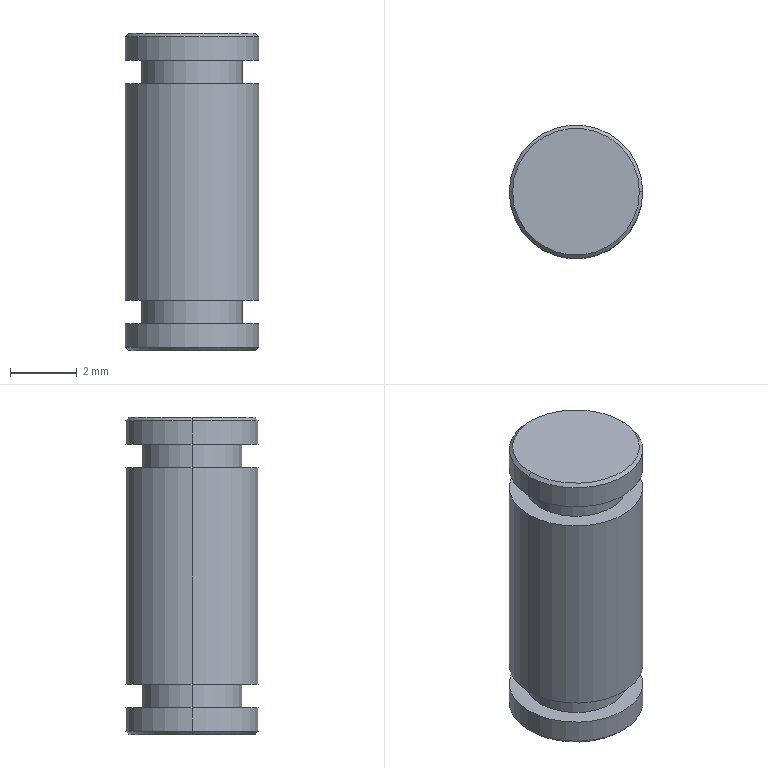Component | SolidWorks | JR-PL-JD-08ConnectingRodPin-1 | 1 solid | 20 faces | box 4 x 4 x 9.5 mm | volume 112 mm3 | cylinder 10 | plane 6 | cone 4 | commonest cylinder face diameters 4 x6 3 x4
build123d program:
from build123d import *

# Parameters (mm, degrees)
CHAMFER1_SIZE = 0.1


with BuildPart() as part:
    # Sketch1 → Revolve1 (revolve)
    with BuildSketch(Plane.XY, mode=Mode.PRIVATE) as revolve1_sk:
        Polygon((0, 0), (0, 2), (0.8, 2), (0.8, 1.5), (1.5, 1.5), (1.5, 2), (8, 2), (8, 1.5), (8.7, 1.5), (8.7, 2), (9.5, 2), (9.5, 0), align=None)
    revolve(revolve1_sk.sketch.rotate(Axis((0, 0, 0), (1, 0, 0)), 90), axis=Axis((0, 0, 0), (1, 0, 0)))

    # Chamfer1
    chamfer1_edges = [part.edges().sort_by_distance(p)[0] for p in [
        (0, 0, -2),
        (9.5, 0, -2),
    ]]
    chamfer(chamfer1_edges, length=CHAMFER1_SIZE)


solid = part.part

# Placed as in the assembly
solid = solid.moved(Location((25.957, 24.823, 72.52), (0, 90, 0)))
STEP:
#1=CARTESIAN_POINT('',(0.9471,0.9773,2.481));
#2=VERTEX_POINT('',#1);
#3=CARTESIAN_POINT('',(1.097,0.9773,2.481));
#4=VERTEX_POINT('',#3);
#5=CARTESIAN_POINT('',(1.022,0.9773,2.481));
#6=DIRECTION('',(0.,0.,-1.));
#7=DIRECTION('',(1.,0.,0.));
#8=AXIS2_PLACEMENT_3D('',#5,#6,#7);
#9=CIRCLE('',#8,0.0748);
#10=EDGE_CURVE('',#2,#4,#9,.T.);
#11=ORIENTED_EDGE('',*,*,#10,.F.);
#12=CARTESIAN_POINT('',(0.9432,0.9773,2.485));
#13=VERTEX_POINT('',#12);
#14=CARTESIAN_POINT('',(0.9471,0.9773,2.481));
#15=DIRECTION('',(-0.7071,0.,0.7071));
#16=VECTOR('',#15,39.37);
#17=LINE('',#14,#16);
#18=EDGE_CURVE('',#2,#13,#17,.T.);
#19=ORIENTED_EDGE('',*,*,#18,.T.);
#20=CARTESIAN_POINT('',(1.101,0.9773,2.485));
#21=VERTEX_POINT('',#20);
#22=CARTESIAN_POINT('',(1.022,0.9773,2.485));
#23=DIRECTION('',(-0.,-0.,1.));
#24=DIRECTION('',(1.,0.,0.));
#25=AXIS2_PLACEMENT_3D('',#22,#23,#24);
#26=CIRCLE('',#25,0.07874);
#27=EDGE_CURVE('',#21,#13,#26,.T.);
#28=ORIENTED_EDGE('',*,*,#27,.F.);
#29=CARTESIAN_POINT('',(1.097,0.9773,2.481));
#30=DIRECTION('',(0.7071,-0.,0.7071));
#31=VECTOR('',#30,39.37);
#32=LINE('',#29,#31);
#33=EDGE_CURVE('',#4,#21,#32,.T.);
#34=ORIENTED_EDGE('',*,*,#33,.F.);
#35=EDGE_LOOP('',(#11,#19,#28,#34));
#36=FACE_OUTER_BOUND('',#35,.T.);
#37=CARTESIAN_POINT('',(1.022,0.9773,2.481));
#38=DIRECTION('',(-0.,-0.,1.));
#39=DIRECTION('',(1.,0.,0.));
#40=AXIS2_PLACEMENT_3D('',#37,#38,#39);
#41=CONICAL_SURFACE('',#40,0.0748,0.7854);
#42=ADVANCED_FACE('',(#36),#41,.T.);
#43=CARTESIAN_POINT('',(1.097,0.9773,2.855));
#44=VERTEX_POINT('',#43);
#45=CARTESIAN_POINT('',(0.9471,0.9773,2.855));
#46=VERTEX_POINT('',#45);
#47=CARTESIAN_POINT('',(1.022,0.9773,2.855));
#48=DIRECTION('',(-0.,-0.,1.));
#49=DIRECTION('',(-1.,0.,0.));
#50=AXIS2_PLACEMENT_3D('',#47,#48,#49);
#51=CIRCLE('',#50,0.0748);
#52=EDGE_CURVE('',#44,#46,#51,.T.);
#53=ORIENTED_EDGE('',*,*,#52,.F.);
#54=CARTESIAN_POINT('',(1.101,0.9773,2.851));
#55=VERTEX_POINT('',#54);
#56=CARTESIAN_POINT('',(1.101,0.9773,2.851));
#57=DIRECTION('',(0.7071,0.,-0.7071));
#58=VECTOR('',#57,39.37);
#59=LINE('',#56,#58);
#60=EDGE_CURVE('',#44,#55,#59,.T.);
#61=ORIENTED_EDGE('',*,*,#60,.T.);
#62=CARTESIAN_POINT('',(0.9432,0.9773,2.851));
#63=VERTEX_POINT('',#62);
#64=CARTESIAN_POINT('',(1.022,0.9773,2.851));
#65=DIRECTION('',(0.,0.,-1.));
#66=DIRECTION('',(-1.,0.,0.));
#67=AXIS2_PLACEMENT_3D('',#64,#65,#66);
#68=CIRCLE('',#67,0.07874);
#69=EDGE_CURVE('',#63,#55,#68,.T.);
#70=ORIENTED_EDGE('',*,*,#69,.F.);
#71=CARTESIAN_POINT('',(0.9432,0.9773,2.851));
#72=DIRECTION('',(-0.7071,0.,-0.7071));
#73=VECTOR('',#72,39.37);
#74=LINE('',#71,#73);
#75=EDGE_CURVE('',#46,#63,#74,.T.);
#76=ORIENTED_EDGE('',*,*,#75,.F.);
#77=EDGE_LOOP('',(#53,#61,#70,#76));
#78=FACE_OUTER_BOUND('',#77,.T.);
#79=CARTESIAN_POINT('',(1.022,0.9773,2.851));
#80=DIRECTION('',(0.,0.,-1.));
#81=DIRECTION('',(-1.,0.,0.));
#82=AXIS2_PLACEMENT_3D('',#79,#80,#81);
#83=CONICAL_SURFACE('',#82,0.07874,0.7854);
#84=ADVANCED_FACE('',(#78),#83,.T.);
#85=ORIENTED_EDGE('',*,*,#69,.T.);
#86=CARTESIAN_POINT('',(1.101,0.9773,2.824));
#87=VERTEX_POINT('',#86);
#88=CARTESIAN_POINT('',(1.101,0.9773,2.481));
#89=DIRECTION('',(0.,0.,-1.));
#90=VECTOR('',#89,39.37);
#91=LINE('',#88,#90);
#92=EDGE_CURVE('',#55,#87,#91,.T.);
#93=ORIENTED_EDGE('',*,*,#92,.T.);
#94=CARTESIAN_POINT('',(0.9432,0.9773,2.824));
#95=VERTEX_POINT('',#94);
#96=CARTESIAN_POINT('',(1.022,0.9773,2.824));
#97=DIRECTION('',(0.,0.,-1.));
#98=DIRECTION('',(-1.,0.,0.));
#99=AXIS2_PLACEMENT_3D('',#96,#97,#98);
#100=CIRCLE('',#99,0.07874);
#101=EDGE_CURVE('',#95,#87,#100,.T.);
#102=ORIENTED_EDGE('',*,*,#101,.F.);
#103=CARTESIAN_POINT('',(0.9432,0.9773,2.481));
#104=DIRECTION('',(0.,0.,-1.));
#105=VECTOR('',#104,39.37);
#106=LINE('',#103,#105);
#107=EDGE_CURVE('',#63,#95,#106,.T.);
#108=ORIENTED_EDGE('',*,*,#107,.F.);
#109=EDGE_LOOP('',(#85,#93,#102,#108));
#110=FACE_OUTER_BOUND('',#109,.T.);
#111=CARTESIAN_POINT('',(1.022,0.9773,2.481));
#112=DIRECTION('',(0.,0.,-1.));
#113=DIRECTION('',(-1.,0.,0.));
#114=AXIS2_PLACEMENT_3D('',#111,#112,#113);
#115=CYLINDRICAL_SURFACE('',#114,0.07874);
#116=ADVANCED_FACE('',(#110),#115,.T.);
#117=CARTESIAN_POINT('',(0.9629,0.9773,2.824));
#118=VERTEX_POINT('',#117);
#119=CARTESIAN_POINT('',(1.081,0.9773,2.824));
#120=VERTEX_POINT('',#119);
#121=CARTESIAN_POINT('',(1.022,0.9773,2.824));
#122=DIRECTION('',(0.,0.,-1.));
#123=DIRECTION('',(-1.,0.,0.));
#124=AXIS2_PLACEMENT_3D('',#121,#122,#123);
#125=CIRCLE('',#124,0.05906);
#126=EDGE_CURVE('',#118,#120,#125,.T.);
#127=ORIENTED_EDGE('',*,*,#126,.T.);
#128=CARTESIAN_POINT('',(1.081,0.9773,2.796));
#129=VERTEX_POINT('',#128);
#130=CARTESIAN_POINT('',(1.081,0.9773,2.481));
#131=DIRECTION('',(0.,0.,-1.));
#132=VECTOR('',#131,39.37);
#133=LINE('',#130,#132);
#134=EDGE_CURVE('',#120,#129,#133,.T.);
#135=ORIENTED_EDGE('',*,*,#134,.T.);
#136=CARTESIAN_POINT('',(0.9629,0.9773,2.796));
#137=VERTEX_POINT('',#136);
#138=CARTESIAN_POINT('',(1.022,0.9773,2.796));
#139=DIRECTION('',(0.,0.,-1.));
#140=DIRECTION('',(-1.,0.,0.));
#141=AXIS2_PLACEMENT_3D('',#138,#139,#140);
#142=CIRCLE('',#141,0.05906);
#143=EDGE_CURVE('',#137,#129,#142,.T.);
#144=ORIENTED_EDGE('',*,*,#143,.F.);
#145=CARTESIAN_POINT('',(0.9629,0.9773,2.481));
#146=DIRECTION('',(0.,0.,-1.));
#147=VECTOR('',#146,39.37);
#148=LINE('',#145,#147);
#149=EDGE_CURVE('',#118,#137,#148,.T.);
#150=ORIENTED_EDGE('',*,*,#149,.F.);
#151=EDGE_LOOP('',(#127,#135,#144,#150));
#152=FACE_OUTER_BOUND('',#151,.T.);
#153=CARTESIAN_POINT('',(1.022,0.9773,2.481));
#154=DIRECTION('',(0.,0.,-1.));
#155=DIRECTION('',(-1.,0.,0.));
#156=AXIS2_PLACEMENT_3D('',#153,#154,#155);
#157=CYLINDRICAL_SURFACE('',#156,0.05906);
#158=ADVANCED_FACE('',(#152),#157,.T.);
#159=CARTESIAN_POINT('',(0.9432,0.9773,2.796));
#160=VERTEX_POINT('',#159);
#161=CARTESIAN_POINT('',(1.101,0.9773,2.796));
#162=VERTEX_POINT('',#161);
#163=CARTESIAN_POINT('',(1.022,0.9773,2.796));
#164=DIRECTION('',(0.,0.,-1.));
#165=DIRECTION('',(-1.,0.,0.));
#166=AXIS2_PLACEMENT_3D('',#163,#164,#165);
#167=CIRCLE('',#166,0.07874);
#168=EDGE_CURVE('',#160,#162,#167,.T.);
#169=ORIENTED_EDGE('',*,*,#168,.T.);
#170=CARTESIAN_POINT('',(1.101,0.9773,2.54));
#171=VERTEX_POINT('',#170);
#172=CARTESIAN_POINT('',(1.101,0.9773,2.481));
#173=DIRECTION('',(0.,0.,-1.));
#174=VECTOR('',#173,39.37);
#175=LINE('',#172,#174);
#176=EDGE_CURVE('',#162,#171,#175,.T.);
#177=ORIENTED_EDGE('',*,*,#176,.T.);
#178=CARTESIAN_POINT('',(0.9432,0.9773,2.54));
#179=VERTEX_POINT('',#178);
#180=CARTESIAN_POINT('',(1.022,0.9773,2.54));
#181=DIRECTION('',(0.,0.,-1.));
#182=DIRECTION('',(-1.,0.,0.));
#183=AXIS2_PLACEMENT_3D('',#180,#181,#182);
#184=CIRCLE('',#183,0.07874);
#185=EDGE_CURVE('',#179,#171,#184,.T.);
#186=ORIENTED_EDGE('',*,*,#185,.F.);
#187=CARTESIAN_POINT('',(0.9432,0.9773,2.481));
#188=DIRECTION('',(0.,0.,-1.));
#189=VECTOR('',#188,39.37);
#190=LINE('',#187,#189);
#191=EDGE_CURVE('',#160,#179,#190,.T.);
#192=ORIENTED_EDGE('',*,*,#191,.F.);
#193=EDGE_LOOP('',(#169,#177,#186,#192));
#194=FACE_OUTER_BOUND('',#193,.T.);
#195=CARTESIAN_POINT('',(1.022,0.9773,2.481));
#196=DIRECTION('',(0.,0.,-1.));
#197=DIRECTION('',(-1.,0.,0.));
#198=AXIS2_PLACEMENT_3D('',#195,#196,#197);
#199=CYLINDRICAL_SURFACE('',#198,0.07874);
#200=ADVANCED_FACE('',(#194),#199,.T.);
#201=CARTESIAN_POINT('',(0.9629,0.9773,2.54));
#202=VERTEX_POINT('',#201);
#203=CARTESIAN_POINT('',(1.081,0.9773,2.54));
#204=VERTEX_POINT('',#203);
#205=CARTESIAN_POINT('',(1.022,0.9773,2.54));
#206=DIRECTION('',(0.,0.,-1.));
#207=DIRECTION('',(-1.,0.,0.));
#208=AXIS2_PLACEMENT_3D('',#205,#206,#207);
#209=CIRCLE('',#208,0.05906);
#210=EDGE_CURVE('',#202,#204,#209,.T.);
#211=ORIENTED_EDGE('',*,*,#210,.T.);
#212=CARTESIAN_POINT('',(1.081,0.9773,2.513));
#213=VERTEX_POINT('',#212);
#214=CARTESIAN_POINT('',(1.081,0.9773,2.481));
#215=DIRECTION('',(0.,0.,-1.));
#216=VECTOR('',#215,39.37);
#217=LINE('',#214,#216);
#218=EDGE_CURVE('',#204,#213,#217,.T.);
#219=ORIENTED_EDGE('',*,*,#218,.T.);
#220=CARTESIAN_POINT('',(0.9629,0.9773,2.513));
#221=VERTEX_POINT('',#220);
#222=CARTESIAN_POINT('',(1.022,0.9773,2.513));
#223=DIRECTION('',(0.,0.,-1.));
#224=DIRECTION('',(-1.,0.,0.));
#225=AXIS2_PLACEMENT_3D('',#222,#223,#224);
#226=CIRCLE('',#225,0.05906);
#227=EDGE_CURVE('',#221,#213,#226,.T.);
#228=ORIENTED_EDGE('',*,*,#227,.F.);
#229=CARTESIAN_POINT('',(0.9629,0.9773,2.481));
#230=DIRECTION('',(0.,0.,-1.));
#231=VECTOR('',#230,39.37);
#232=LINE('',#229,#231);
#233=EDGE_CURVE('',#202,#221,#232,.T.);
#234=ORIENTED_EDGE('',*,*,#233,.F.);
#235=EDGE_LOOP('',(#211,#219,#228,#234));
#236=FACE_OUTER_BOUND('',#235,.T.);
#237=CARTESIAN_POINT('',(1.022,0.9773,2.481));
#238=DIRECTION('',(0.,0.,-1.));
#239=DIRECTION('',(-1.,0.,0.));
#240=AXIS2_PLACEMENT_3D('',#237,#238,#239);
#241=CYLINDRICAL_SURFACE('',#240,0.05906);
#242=ADVANCED_FACE('',(#236),#241,.T.);
#243=CARTESIAN_POINT('',(0.9432,0.9773,2.513));
#244=VERTEX_POINT('',#243);
#245=CARTESIAN_POINT('',(1.101,0.9773,2.513));
#246=VERTEX_POINT('',#245);
#247=CARTESIAN_POINT('',(1.022,0.9773,2.513));
#248=DIRECTION('',(0.,0.,-1.));
#249=DIRECTION('',(-1.,0.,0.));
#250=AXIS2_PLACEMENT_3D('',#247,#248,#249);
#251=CIRCLE('',#250,0.07874);
#252=EDGE_CURVE('',#244,#246,#251,.T.);
#253=ORIENTED_EDGE('',*,*,#252,.T.);
#254=CARTESIAN_POINT('',(1.101,0.9773,2.481));
#255=DIRECTION('',(0.,0.,-1.));
#256=VECTOR('',#255,39.37);
#257=LINE('',#254,#256);
#258=EDGE_CURVE('',#246,#21,#257,.T.);
#259=ORIENTED_EDGE('',*,*,#258,.T.);
#260=ORIENTED_EDGE('',*,*,#27,.T.);
#261=CARTESIAN_POINT('',(0.9432,0.9773,2.481));
#262=DIRECTION('',(0.,0.,-1.));
#263=VECTOR('',#262,39.37);
#264=LINE('',#261,#263);
#265=EDGE_CURVE('',#244,#13,#264,.T.);
#266=ORIENTED_EDGE('',*,*,#265,.F.);
#267=EDGE_LOOP('',(#253,#259,#260,#266));
#268=FACE_OUTER_BOUND('',#267,.T.);
#269=CARTESIAN_POINT('',(1.022,0.9773,2.481));
#270=DIRECTION('',(0.,0.,-1.));
#271=DIRECTION('',(-1.,0.,0.));
#272=AXIS2_PLACEMENT_3D('',#269,#270,#271);
#273=CYLINDRICAL_SURFACE('',#272,0.07874);
#274=ADVANCED_FACE('',(#268),#273,.T.);
#275=CARTESIAN_POINT('',(1.022,0.9773,2.481));
#276=DIRECTION('',(0.,0.,-1.));
#277=DIRECTION('',(1.,0.,0.));
#278=AXIS2_PLACEMENT_3D('',#275,#276,#277);
#279=CIRCLE('',#278,0.0748);
#280=EDGE_CURVE('',#4,#2,#279,.T.);
#281=ORIENTED_EDGE('',*,*,#280,.T.);
#282=ORIENTED_EDGE('',*,*,#10,.T.);
#283=EDGE_LOOP('',(#281,#282));
#284=FACE_OUTER_BOUND('',#283,.T.);
#285=CARTESIAN_POINT('',(1.022,0.9773,2.481));
#286=DIRECTION('',(-0.,-0.,1.));
#287=DIRECTION('',(1.,-0.,0.));
#288=AXIS2_PLACEMENT_3D('',#285,#286,#287);
#289=PLANE('',#288);
#290=ADVANCED_FACE('',(#284),#289,.F.);
#291=ORIENTED_EDGE('',*,*,#258,.F.);
#292=CARTESIAN_POINT('',(1.022,0.9773,2.513));
#293=DIRECTION('',(0.,0.,-1.));
#294=DIRECTION('',(-1.,0.,0.));
#295=AXIS2_PLACEMENT_3D('',#292,#293,#294);
#296=CIRCLE('',#295,0.07874);
#297=EDGE_CURVE('',#246,#244,#296,.T.);
#298=ORIENTED_EDGE('',*,*,#297,.T.);
#299=ORIENTED_EDGE('',*,*,#265,.T.);
#300=CARTESIAN_POINT('',(1.022,0.9773,2.485));
#301=DIRECTION('',(-0.,-0.,1.));
#302=DIRECTION('',(1.,0.,0.));
#303=AXIS2_PLACEMENT_3D('',#300,#301,#302);
#304=CIRCLE('',#303,0.07874);
#305=EDGE_CURVE('',#13,#21,#304,.T.);
#306=ORIENTED_EDGE('',*,*,#305,.T.);
#307=EDGE_LOOP('',(#291,#298,#299,#306));
#308=FACE_OUTER_BOUND('',#307,.T.);
#309=CARTESIAN_POINT('',(1.022,0.9773,2.481));
#310=DIRECTION('',(0.,0.,-1.));
#311=DIRECTION('',(-1.,0.,0.));
#312=AXIS2_PLACEMENT_3D('',#309,#310,#311);
#313=CYLINDRICAL_SURFACE('',#312,0.07874);
#314=ADVANCED_FACE('',(#308),#313,.T.);
#315=ORIENTED_EDGE('',*,*,#252,.F.);
#316=ORIENTED_EDGE('',*,*,#297,.F.);
#317=EDGE_LOOP('',(#315,#316));
#318=FACE_OUTER_BOUND('',#317,.T.);
#319=ORIENTED_EDGE('',*,*,#227,.T.);
#320=CARTESIAN_POINT('',(1.022,0.9773,2.513));
#321=DIRECTION('',(0.,0.,-1.));
#322=DIRECTION('',(-1.,0.,0.));
#323=AXIS2_PLACEMENT_3D('',#320,#321,#322);
#324=CIRCLE('',#323,0.05906);
#325=EDGE_CURVE('',#213,#221,#324,.T.);
#326=ORIENTED_EDGE('',*,*,#325,.T.);
#327=EDGE_LOOP('',(#319,#326));
#328=FACE_BOUND('',#327,.T.);
#329=CARTESIAN_POINT('',(1.022,1.056,2.513));
#330=DIRECTION('',(0.,0.,-1.));
#331=DIRECTION('',(-1.,0.,-0.));
#332=AXIS2_PLACEMENT_3D('',#329,#330,#331);
#333=PLANE('',#332);
#334=ADVANCED_FACE('',(#318,#328),#333,.F.);
#335=ORIENTED_EDGE('',*,*,#218,.F.);
#336=CARTESIAN_POINT('',(1.022,0.9773,2.54));
#337=DIRECTION('',(0.,0.,-1.));
#338=DIRECTION('',(-1.,0.,0.));
#339=AXIS2_PLACEMENT_3D('',#336,#337,#338);
#340=CIRCLE('',#339,0.05906);
#341=EDGE_CURVE('',#204,#202,#340,.T.);
#342=ORIENTED_EDGE('',*,*,#341,.T.);
#343=ORIENTED_EDGE('',*,*,#233,.T.);
#344=ORIENTED_EDGE('',*,*,#325,.F.);
#345=EDGE_LOOP('',(#335,#342,#343,#344));
#346=FACE_OUTER_BOUND('',#345,.T.);
#347=CARTESIAN_POINT('',(1.022,0.9773,2.481));
#348=DIRECTION('',(0.,0.,-1.));
#349=DIRECTION('',(-1.,0.,0.));
#350=AXIS2_PLACEMENT_3D('',#347,#348,#349);
#351=CYLINDRICAL_SURFACE('',#350,0.05906);
#352=ADVANCED_FACE('',(#346),#351,.T.);
#353=ORIENTED_EDGE('',*,*,#210,.F.);
#354=ORIENTED_EDGE('',*,*,#341,.F.);
#355=EDGE_LOOP('',(#353,#354));
#356=FACE_BOUND('',#355,.T.);
#357=ORIENTED_EDGE('',*,*,#185,.T.);
#358=CARTESIAN_POINT('',(1.022,0.9773,2.54));
#359=DIRECTION('',(0.,0.,-1.));
#360=DIRECTION('',(-1.,0.,0.));
#361=AXIS2_PLACEMENT_3D('',#358,#359,#360);
#362=CIRCLE('',#361,0.07874);
#363=EDGE_CURVE('',#171,#179,#362,.T.);
#364=ORIENTED_EDGE('',*,*,#363,.T.);
#365=EDGE_LOOP('',(#357,#364));
#366=FACE_OUTER_BOUND('',#365,.T.);
#367=CARTESIAN_POINT('',(1.022,1.036,2.54));
#368=DIRECTION('',(-0.,-0.,1.));
#369=DIRECTION('',(1.,-0.,0.));
#370=AXIS2_PLACEMENT_3D('',#367,#368,#369);
#371=PLANE('',#370);
#372=ADVANCED_FACE('',(#356,#366),#371,.F.);
#373=ORIENTED_EDGE('',*,*,#176,.F.);
#374=CARTESIAN_POINT('',(1.022,0.9773,2.796));
#375=DIRECTION('',(0.,0.,-1.));
#376=DIRECTION('',(-1.,0.,0.));
#377=AXIS2_PLACEMENT_3D('',#374,#375,#376);
#378=CIRCLE('',#377,0.07874);
#379=EDGE_CURVE('',#162,#160,#378,.T.);
#380=ORIENTED_EDGE('',*,*,#379,.T.);
#381=ORIENTED_EDGE('',*,*,#191,.T.);
#382=ORIENTED_EDGE('',*,*,#363,.F.);
#383=EDGE_LOOP('',(#373,#380,#381,#382));
#384=FACE_OUTER_BOUND('',#383,.T.);
#385=CARTESIAN_POINT('',(1.022,0.9773,2.481));
#386=DIRECTION('',(0.,0.,-1.));
#387=DIRECTION('',(-1.,0.,0.));
#388=AXIS2_PLACEMENT_3D('',#385,#386,#387);
#389=CYLINDRICAL_SURFACE('',#388,0.07874);
#390=ADVANCED_FACE('',(#384),#389,.T.);
#391=ORIENTED_EDGE('',*,*,#168,.F.);
#392=ORIENTED_EDGE('',*,*,#379,.F.);
#393=EDGE_LOOP('',(#391,#392));
#394=FACE_OUTER_BOUND('',#393,.T.);
#395=ORIENTED_EDGE('',*,*,#143,.T.);
#396=CARTESIAN_POINT('',(1.022,0.9773,2.796));
#397=DIRECTION('',(0.,0.,-1.));
#398=DIRECTION('',(-1.,0.,0.));
#399=AXIS2_PLACEMENT_3D('',#396,#397,#398);
#400=CIRCLE('',#399,0.05906);
#401=EDGE_CURVE('',#129,#137,#400,.T.);
#402=ORIENTED_EDGE('',*,*,#401,.T.);
#403=EDGE_LOOP('',(#395,#402));
#404=FACE_BOUND('',#403,.T.);
#405=CARTESIAN_POINT('',(1.022,1.036,2.796));
#406=DIRECTION('',(0.,0.,-1.));
#407=DIRECTION('',(-1.,0.,-0.));
#408=AXIS2_PLACEMENT_3D('',#405,#406,#407);
#409=PLANE('',#408);
#410=ADVANCED_FACE('',(#394,#404),#409,.F.);
#411=ORIENTED_EDGE('',*,*,#134,.F.);
#412=CARTESIAN_POINT('',(1.022,0.9773,2.824));
#413=DIRECTION('',(0.,0.,-1.));
#414=DIRECTION('',(-1.,0.,0.));
#415=AXIS2_PLACEMENT_3D('',#412,#413,#414);
#416=CIRCLE('',#415,0.05906);
#417=EDGE_CURVE('',#120,#118,#416,.T.);
#418=ORIENTED_EDGE('',*,*,#417,.T.);
#419=ORIENTED_EDGE('',*,*,#149,.T.);
#420=ORIENTED_EDGE('',*,*,#401,.F.);
#421=EDGE_LOOP('',(#411,#418,#419,#420));
#422=FACE_OUTER_BOUND('',#421,.T.);
#423=CARTESIAN_POINT('',(1.022,0.9773,2.481));
#424=DIRECTION('',(0.,0.,-1.));
#425=DIRECTION('',(-1.,0.,0.));
#426=AXIS2_PLACEMENT_3D('',#423,#424,#425);
#427=CYLINDRICAL_SURFACE('',#426,0.05906);
#428=ADVANCED_FACE('',(#422),#427,.T.);
#429=ORIENTED_EDGE('',*,*,#126,.F.);
#430=ORIENTED_EDGE('',*,*,#417,.F.);
#431=EDGE_LOOP('',(#429,#430));
#432=FACE_BOUND('',#431,.T.);
#433=ORIENTED_EDGE('',*,*,#101,.T.);
#434=CARTESIAN_POINT('',(1.022,0.9773,2.824));
#435=DIRECTION('',(0.,0.,-1.));
#436=DIRECTION('',(-1.,0.,0.));
#437=AXIS2_PLACEMENT_3D('',#434,#435,#436);
#438=CIRCLE('',#437,0.07874);
#439=EDGE_CURVE('',#87,#95,#438,.T.);
#440=ORIENTED_EDGE('',*,*,#439,.T.);
#441=EDGE_LOOP('',(#433,#440));
#442=FACE_OUTER_BOUND('',#441,.T.);
#443=CARTESIAN_POINT('',(1.022,1.056,2.824));
#444=DIRECTION('',(-0.,-0.,1.));
#445=DIRECTION('',(1.,-0.,0.));
#446=AXIS2_PLACEMENT_3D('',#443,#444,#445);
#447=PLANE('',#446);
#448=ADVANCED_FACE('',(#432,#442),#447,.F.);
#449=ORIENTED_EDGE('',*,*,#92,.F.);
#450=CARTESIAN_POINT('',(1.022,0.9773,2.851));
#451=DIRECTION('',(0.,0.,-1.));
#452=DIRECTION('',(-1.,0.,0.));
#453=AXIS2_PLACEMENT_3D('',#450,#451,#452);
#454=CIRCLE('',#453,0.07874);
#455=EDGE_CURVE('',#55,#63,#454,.T.);
#456=ORIENTED_EDGE('',*,*,#455,.T.);
#457=ORIENTED_EDGE('',*,*,#107,.T.);
#458=ORIENTED_EDGE('',*,*,#439,.F.);
#459=EDGE_LOOP('',(#449,#456,#457,#458));
#460=FACE_OUTER_BOUND('',#459,.T.);
#461=CARTESIAN_POINT('',(1.022,0.9773,2.481));
#462=DIRECTION('',(0.,0.,-1.));
#463=DIRECTION('',(-1.,0.,0.));
#464=AXIS2_PLACEMENT_3D('',#461,#462,#463);
#465=CYLINDRICAL_SURFACE('',#464,0.07874);
#466=ADVANCED_FACE('',(#460),#465,.T.);
#467=CARTESIAN_POINT('',(1.022,0.9773,2.855));
#468=DIRECTION('',(-0.,-0.,1.));
#469=DIRECTION('',(-1.,0.,0.));
#470=AXIS2_PLACEMENT_3D('',#467,#468,#469);
#471=CIRCLE('',#470,0.0748);
#472=EDGE_CURVE('',#46,#44,#471,.T.);
#473=ORIENTED_EDGE('',*,*,#472,.T.);
#474=ORIENTED_EDGE('',*,*,#52,.T.);
#475=EDGE_LOOP('',(#473,#474));
#476=FACE_OUTER_BOUND('',#475,.T.);
#477=CARTESIAN_POINT('',(1.022,0.9773,2.855));
#478=DIRECTION('',(0.,0.,-1.));
#479=DIRECTION('',(-1.,0.,-0.));
#480=AXIS2_PLACEMENT_3D('',#477,#478,#479);
#481=PLANE('',#480);
#482=ADVANCED_FACE('',(#476),#481,.F.);
#483=ORIENTED_EDGE('',*,*,#60,.F.);
#484=ORIENTED_EDGE('',*,*,#472,.F.);
#485=ORIENTED_EDGE('',*,*,#75,.T.);
#486=ORIENTED_EDGE('',*,*,#455,.F.);
#487=EDGE_LOOP('',(#483,#484,#485,#486));
#488=FACE_OUTER_BOUND('',#487,.T.);
#489=CARTESIAN_POINT('',(1.022,0.9773,2.851));
#490=DIRECTION('',(0.,0.,-1.));
#491=DIRECTION('',(-1.,0.,0.));
#492=AXIS2_PLACEMENT_3D('',#489,#490,#491);
#493=CONICAL_SURFACE('',#492,0.07874,0.7854);
#494=ADVANCED_FACE('',(#488),#493,.T.);
#495=ORIENTED_EDGE('',*,*,#18,.F.);
#496=ORIENTED_EDGE('',*,*,#280,.F.);
#497=ORIENTED_EDGE('',*,*,#33,.T.);
#498=ORIENTED_EDGE('',*,*,#305,.F.);
#499=EDGE_LOOP('',(#495,#496,#497,#498));
#500=FACE_OUTER_BOUND('',#499,.T.);
#501=CARTESIAN_POINT('',(1.022,0.9773,2.481));
#502=DIRECTION('',(-0.,-0.,1.));
#503=DIRECTION('',(1.,0.,0.));
#504=AXIS2_PLACEMENT_3D('',#501,#502,#503);
#505=CONICAL_SURFACE('',#504,0.0748,0.7854);
#506=ADVANCED_FACE('',(#500),#505,.T.);
#507=CLOSED_SHELL('',(#42,#84,#116,#158,#200,#242,#274,#290,#314,#334,#352,#372,#390,#410,#428,#448,#466,#482,#494,#506));
#508=MANIFOLD_SOLID_BREP('',#507);
#509=CARTESIAN_POINT('',(0.,0.,0.));
#510=DIRECTION('',(0.,0.,1.));
#511=DIRECTION('',(1.,0.,0.));
#512=AXIS2_PLACEMENT_3D('',#509,#510,#511);
#513=(LENGTH_UNIT()NAMED_UNIT(*)SI_UNIT($,.METRE.));
#514=LENGTH_MEASURE_WITH_UNIT(LENGTH_MEASURE(0.0254),#513);
#515=DIMENSIONAL_EXPONENTS(1.,0.,0.,0.,0.,0.,0.);
#516=(CONVERSION_BASED_UNIT('',#514)LENGTH_UNIT()NAMED_UNIT(#515));
#517=UNCERTAINTY_MEASURE_WITH_UNIT(LENGTH_MEASURE(0.00001),#516,'','');
#518=(NAMED_UNIT(*)PLANE_ANGLE_UNIT()SI_UNIT($,.RADIAN.));
#519=(NAMED_UNIT(*)SI_UNIT($,.STERADIAN.)SOLID_ANGLE_UNIT());
#520=(GEOMETRIC_REPRESENTATION_CONTEXT(3)GLOBAL_UNCERTAINTY_ASSIGNED_CONTEXT((#517))GLOBAL_UNIT_ASSIGNED_CONTEXT((#516,#518,#519))REPRESENTATION_CONTEXT('',''));
#521=ADVANCED_BREP_SHAPE_REPRESENTATION('',(#508,#512),#520);
#522=COLOUR_RGB('',0.7922,0.8196,0.9333);
#523=FILL_AREA_STYLE_COLOUR('',#522);
#524=FILL_AREA_STYLE('',(#523));
#525=SURFACE_STYLE_FILL_AREA(#524);
#526=SURFACE_SIDE_STYLE('',(#525));
#527=SURFACE_STYLE_USAGE(.BOTH.,#526);
#528=PRESENTATION_STYLE_ASSIGNMENT((#527));
#529=STYLED_ITEM('',(#528),#508);
#530=(LENGTH_UNIT()NAMED_UNIT(*)SI_UNIT($,.METRE.));
#531=LENGTH_MEASURE_WITH_UNIT(LENGTH_MEASURE(0.0254),#530);
#532=DIMENSIONAL_EXPONENTS(1.,0.,0.,0.,0.,0.,0.);
#533=(CONVERSION_BASED_UNIT('',#531)LENGTH_UNIT()NAMED_UNIT(#532));
#534=UNCERTAINTY_MEASURE_WITH_UNIT(LENGTH_MEASURE(0.00001),#533,'','');
#535=(NAMED_UNIT(*)PLANE_ANGLE_UNIT()SI_UNIT($,.RADIAN.));
#536=(NAMED_UNIT(*)SI_UNIT($,.STERADIAN.)SOLID_ANGLE_UNIT());
#537=(GEOMETRIC_REPRESENTATION_CONTEXT(3)GLOBAL_UNCERTAINTY_ASSIGNED_CONTEXT((#534))GLOBAL_UNIT_ASSIGNED_CONTEXT((#533,#535,#536))REPRESENTATION_CONTEXT('',''));
#538=MECHANICAL_DESIGN_GEOMETRIC_PRESENTATION_REPRESENTATION('',(#529),#537);
#539=PRESENTATION_LAYER_ASSIGNMENT('','',(#529));